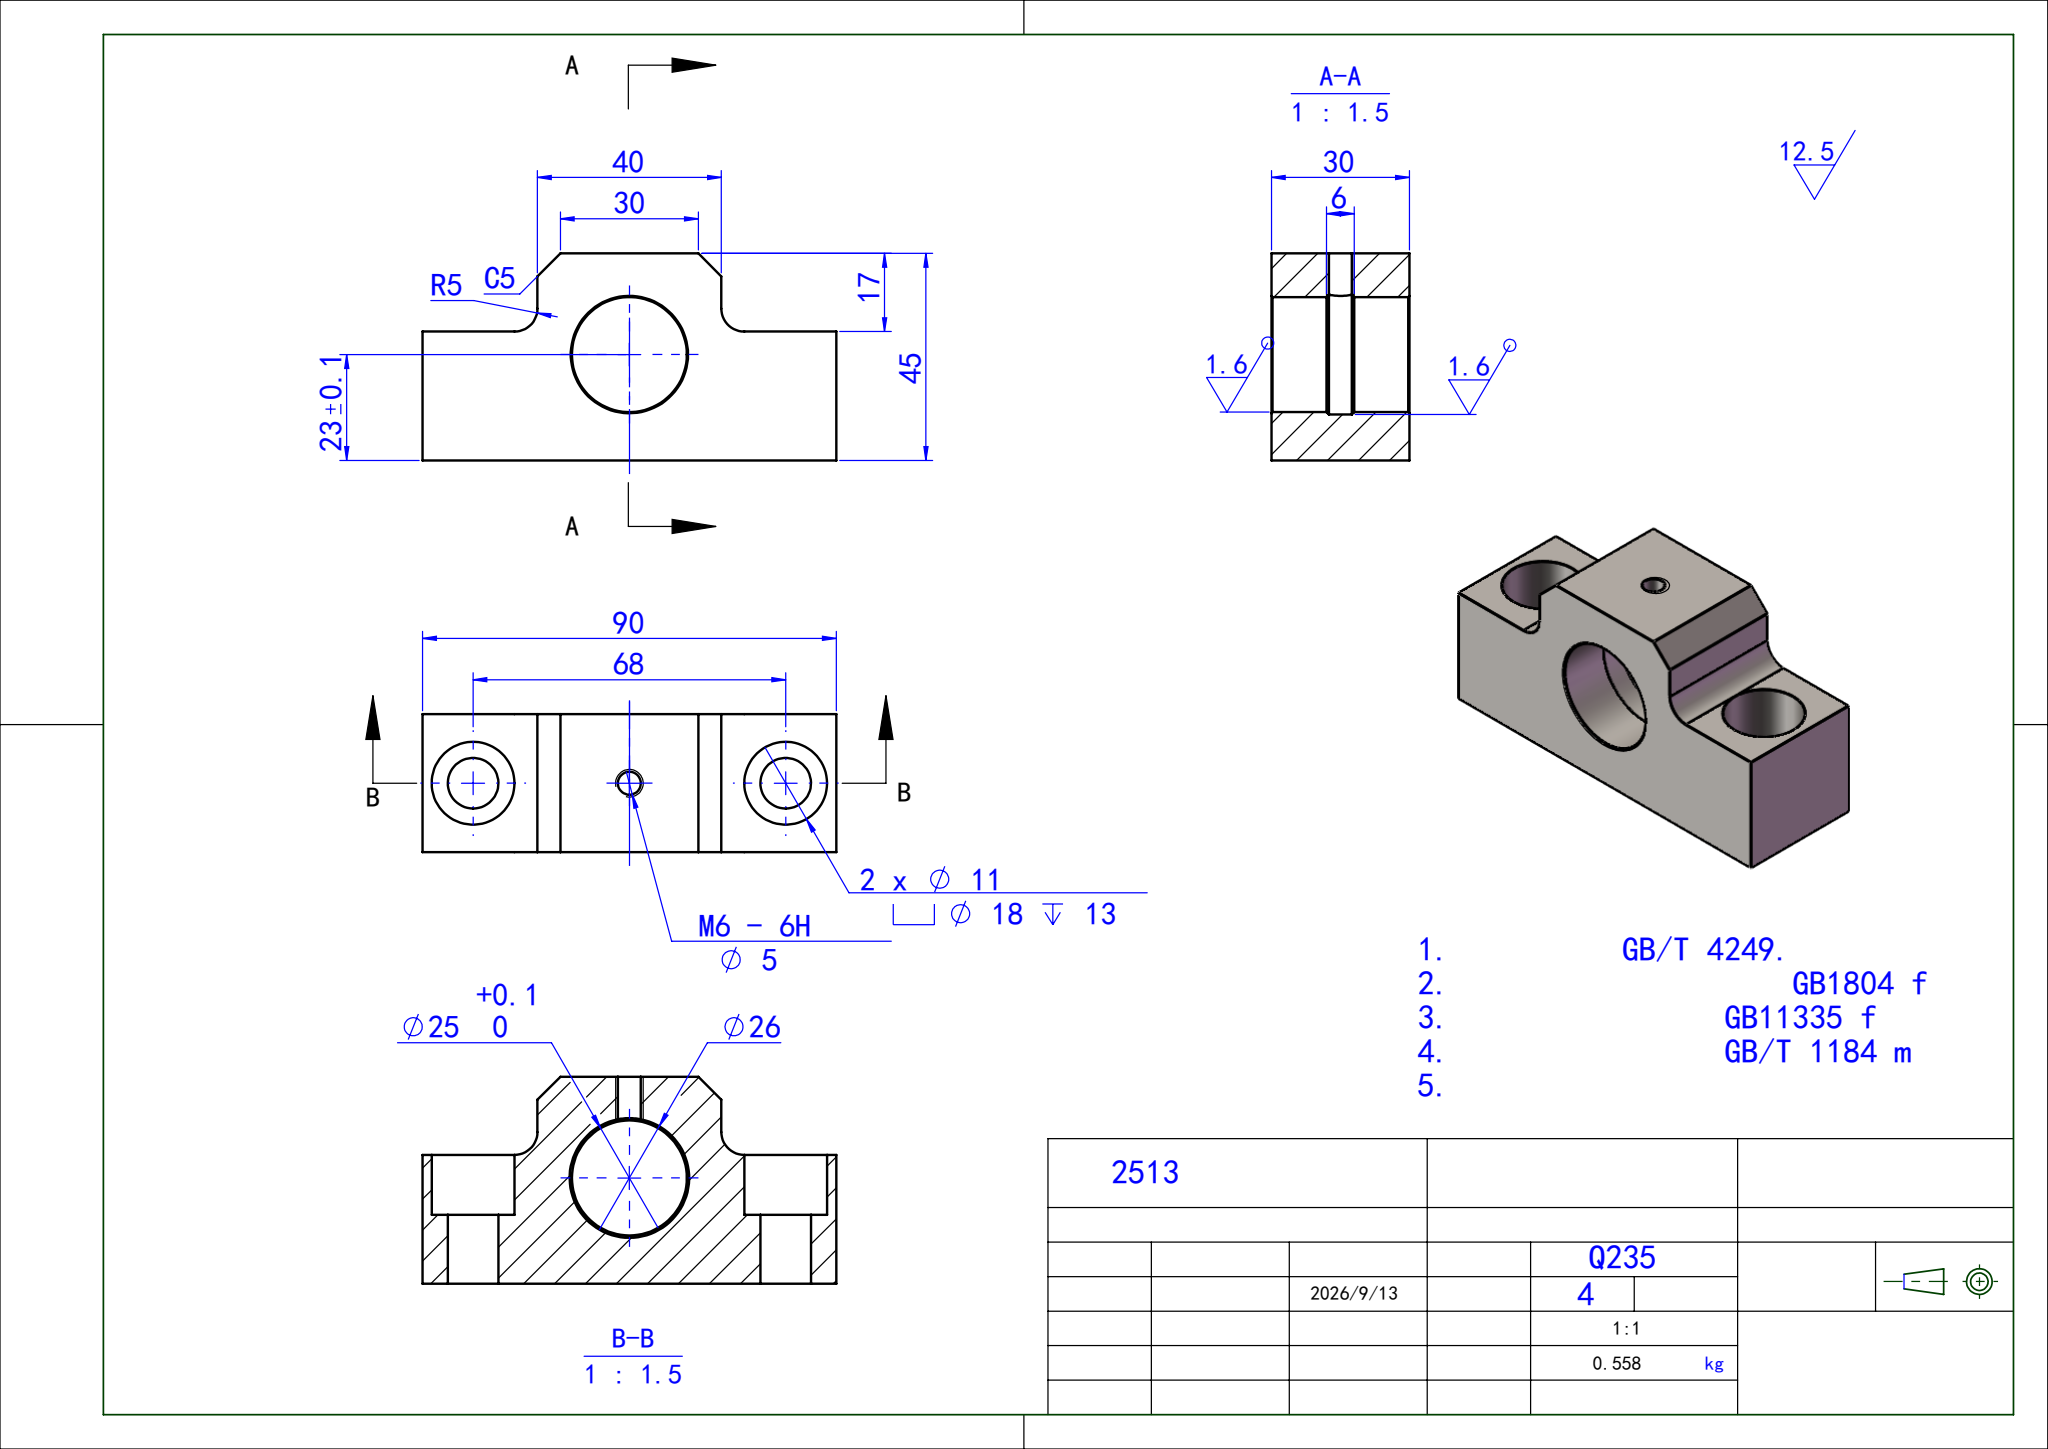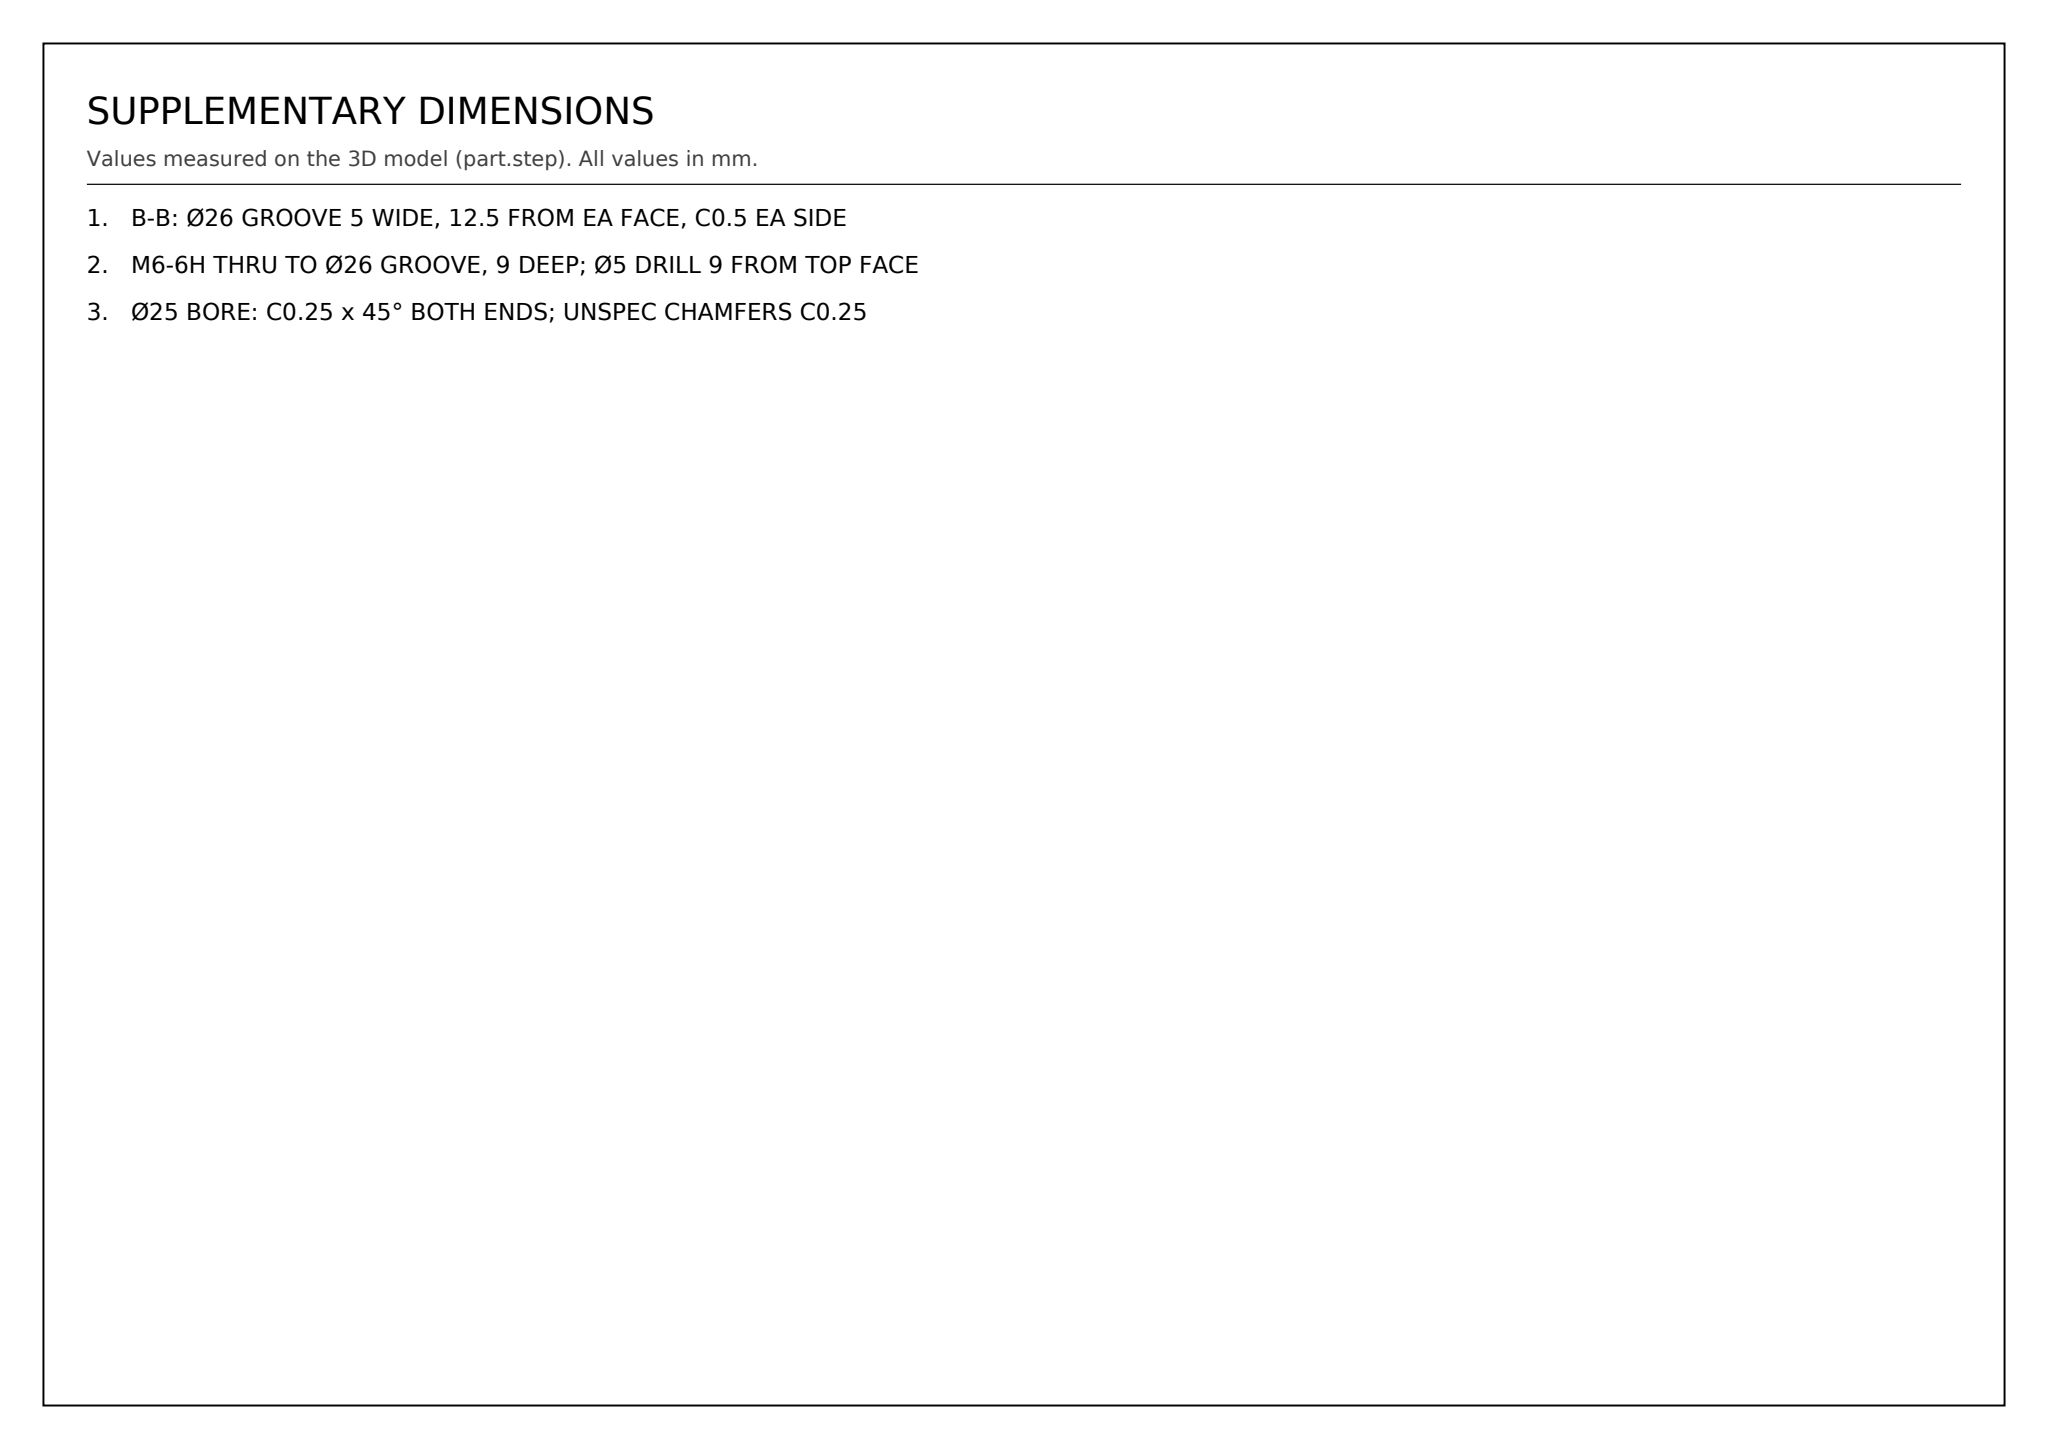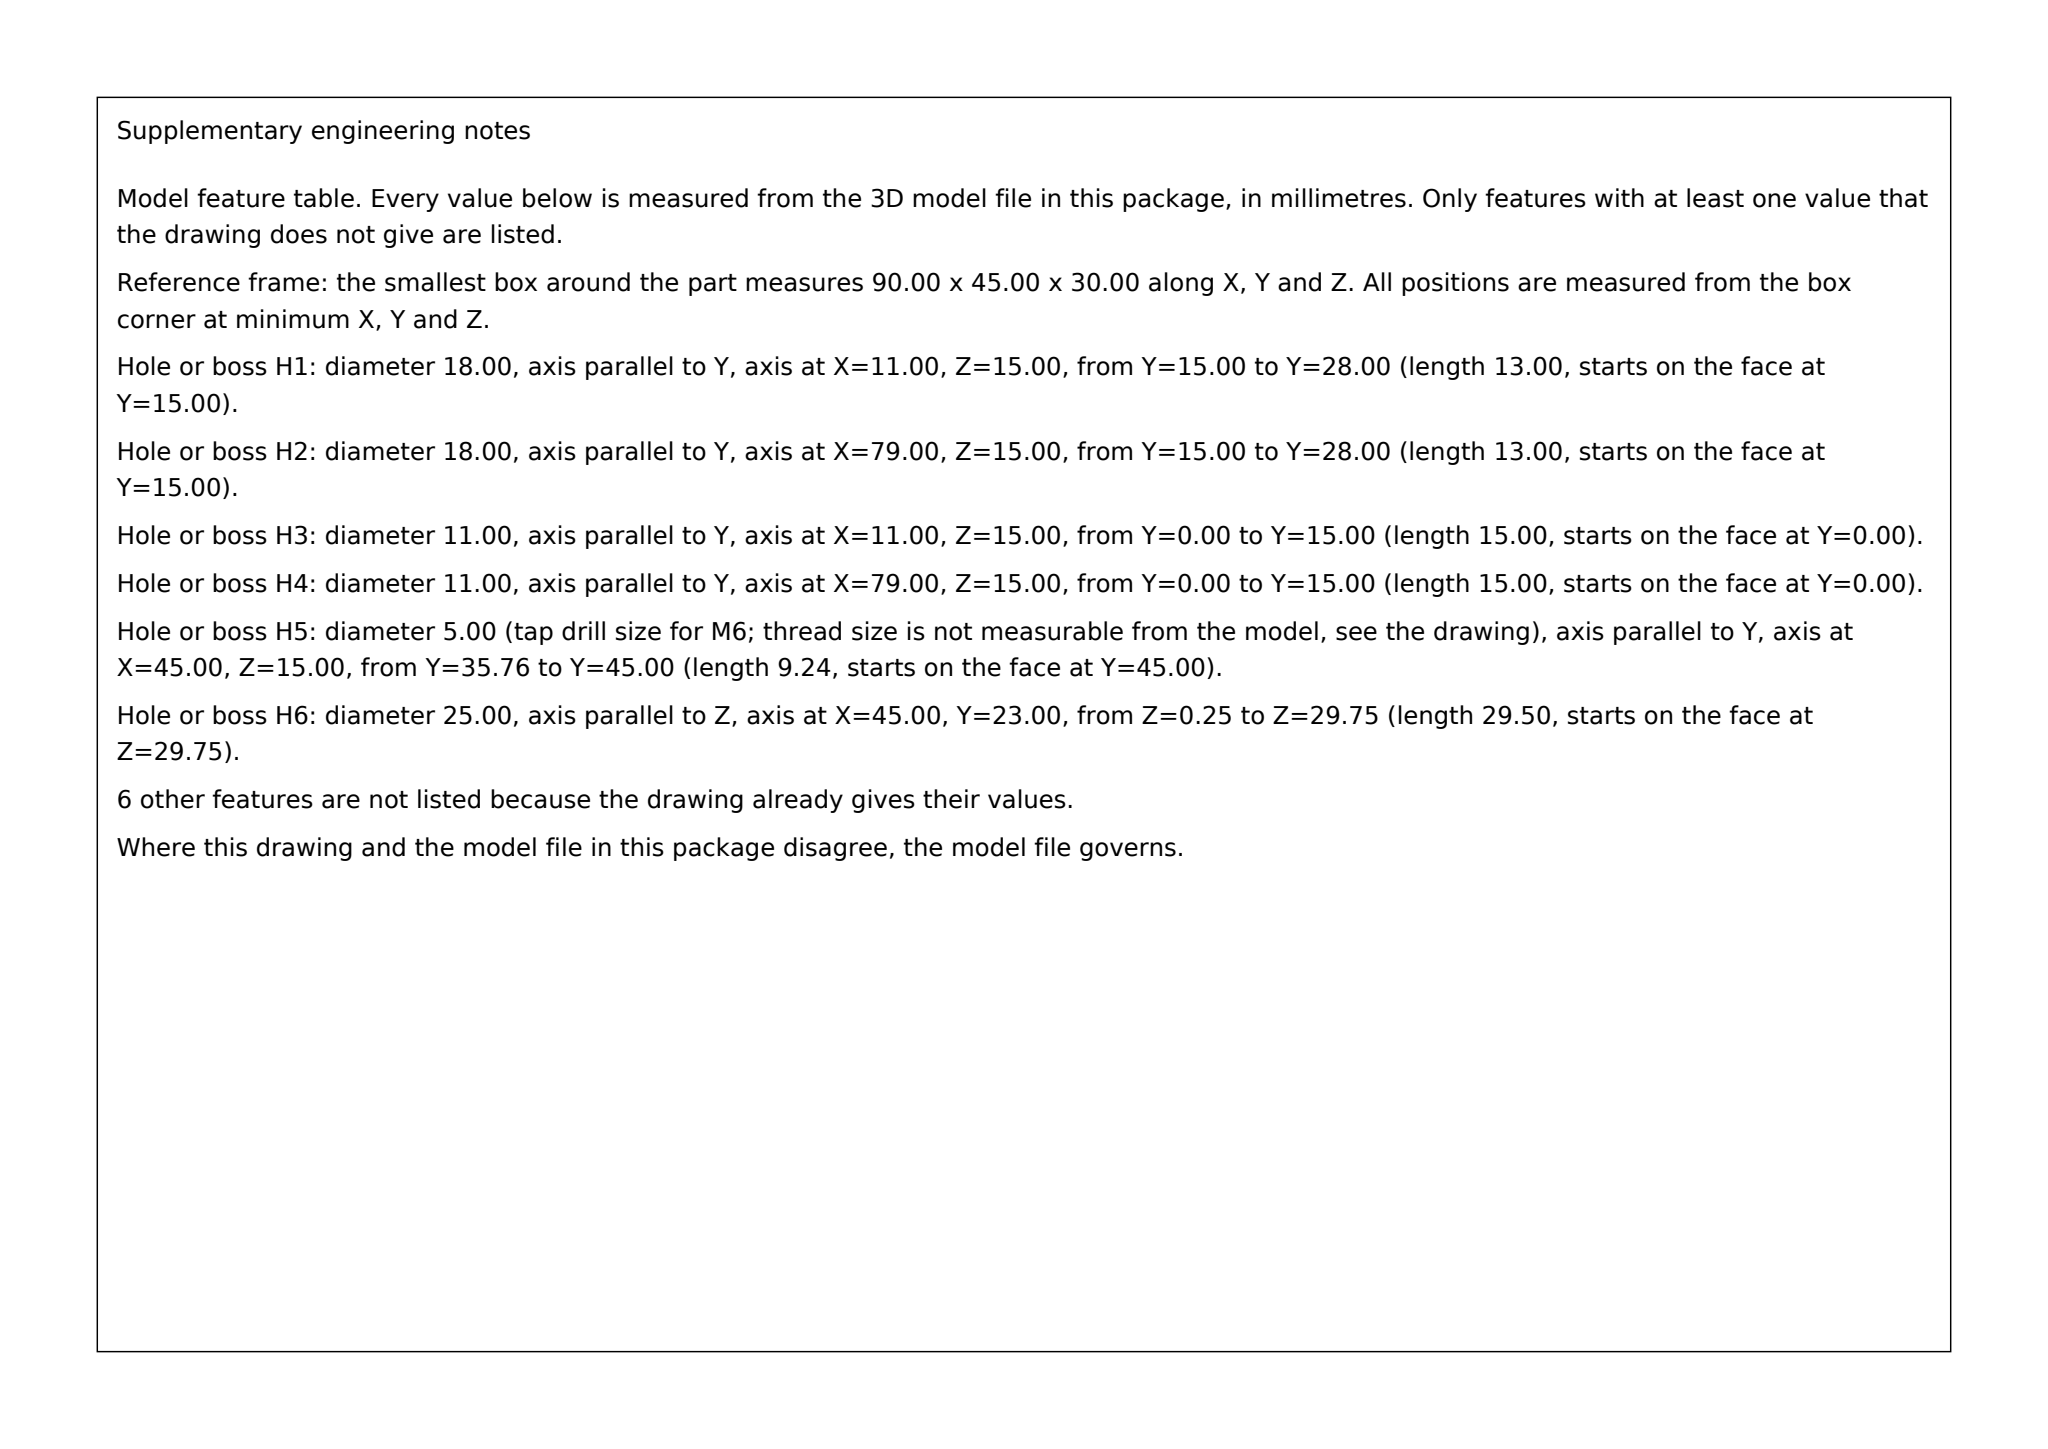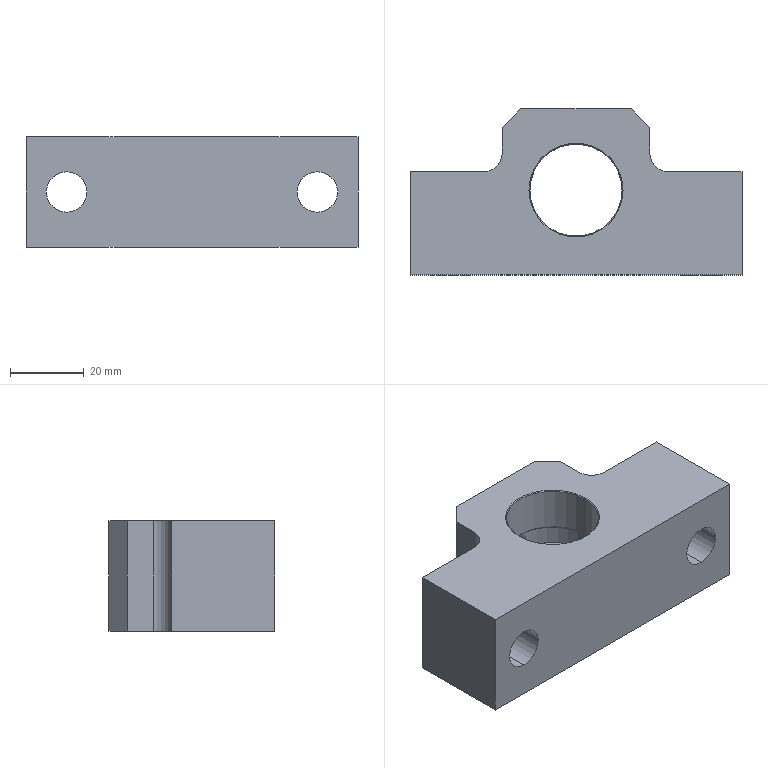Part | SolidWorks | mm | material Q235 | 1 solid | 41 faces | box 90 x 45 x 30 mm | volume 70975 mm3 | cylinder 19 | plane 14 | cone 8 | commonest cylinder face diameters 18 x4 11 x4 25 x4 26 x3 5 x2 10 x2
Drawing notes:
B-B: Ø26 GROOVE 5 WIDE, 12.5 FROM EA FACE, C0.5 EA SIDE | from the solid: Ø26 cyl on bore axis (45,23), axial len 5.0 in 30 thk, flanked by Ø25 cyls 11.75 ea => groove ctrd z12.5-17.5; 90° cones ref Ø26 at groove sides
M6-6H THRU TO Ø26 GROOVE, 9 DEEP; Ø5 DRILL 9 FROM TOP FACE | from the solid: Ø5 cyl along y at x=45,z=15, len 9.24 from top face y=45 (bbox 45 high); breaks into Ø26 groove whose crown is y=23+13=36 => 9 at axis
Ø25 BORE: C0.25 x 45° BOTH ENDS; UNSPEC CHAMFERS C0.25 | from the solid: cones 90° ref Ø25.5 at bore ends; 30 - 2x11.75 - 5 - 2x0.5(groove cones) = 0.5 => 0.25 axial per end, Ø25->Ø25.5